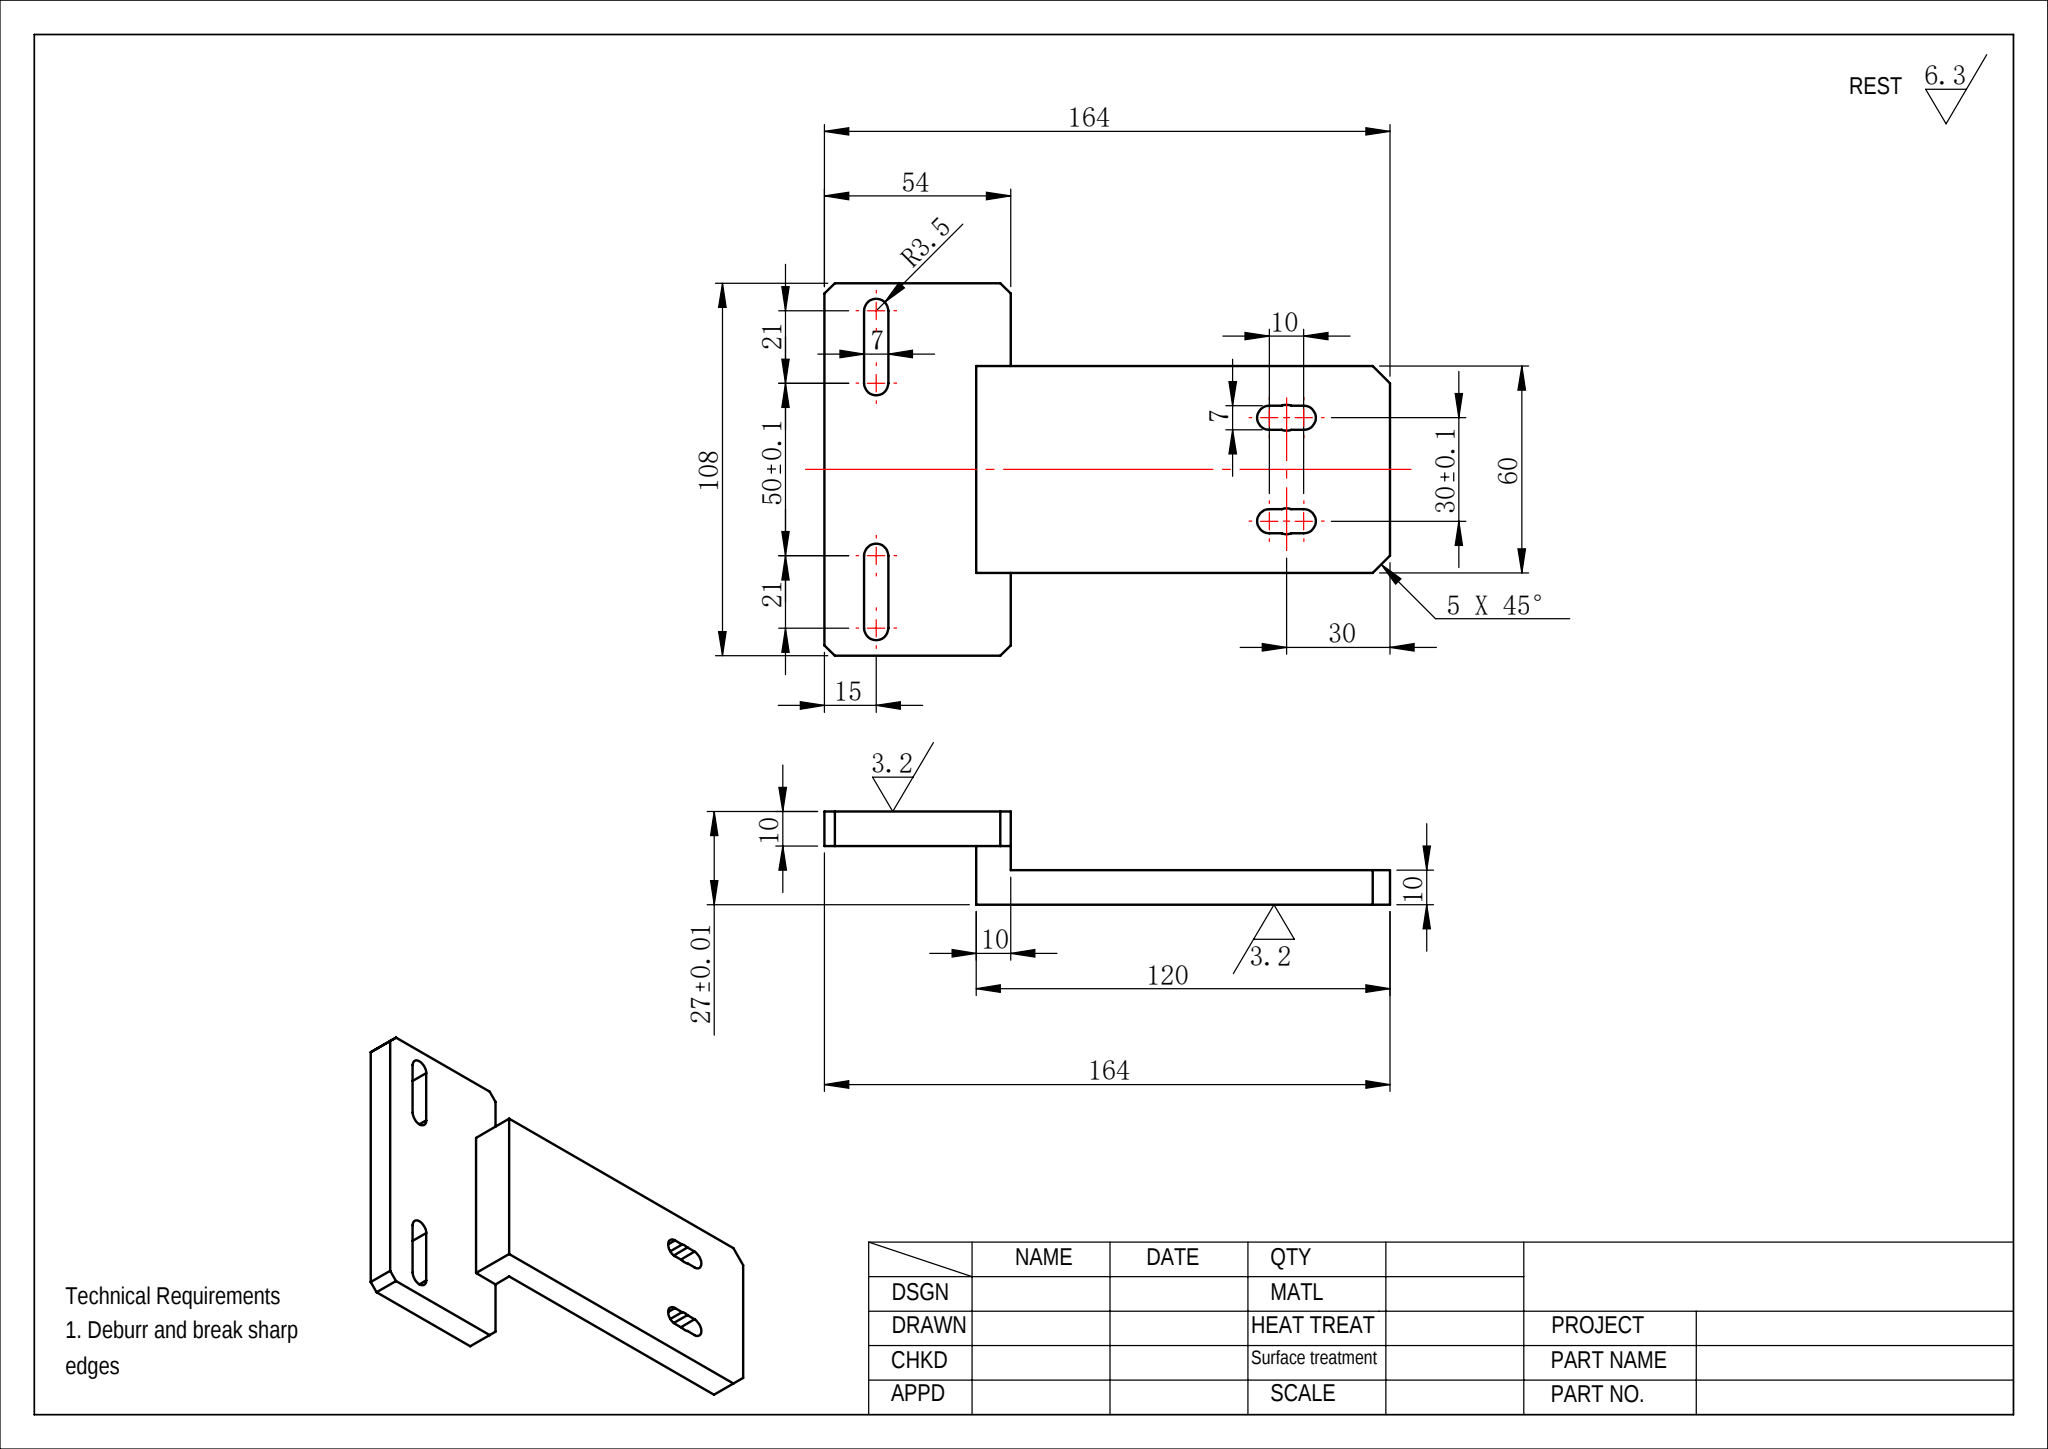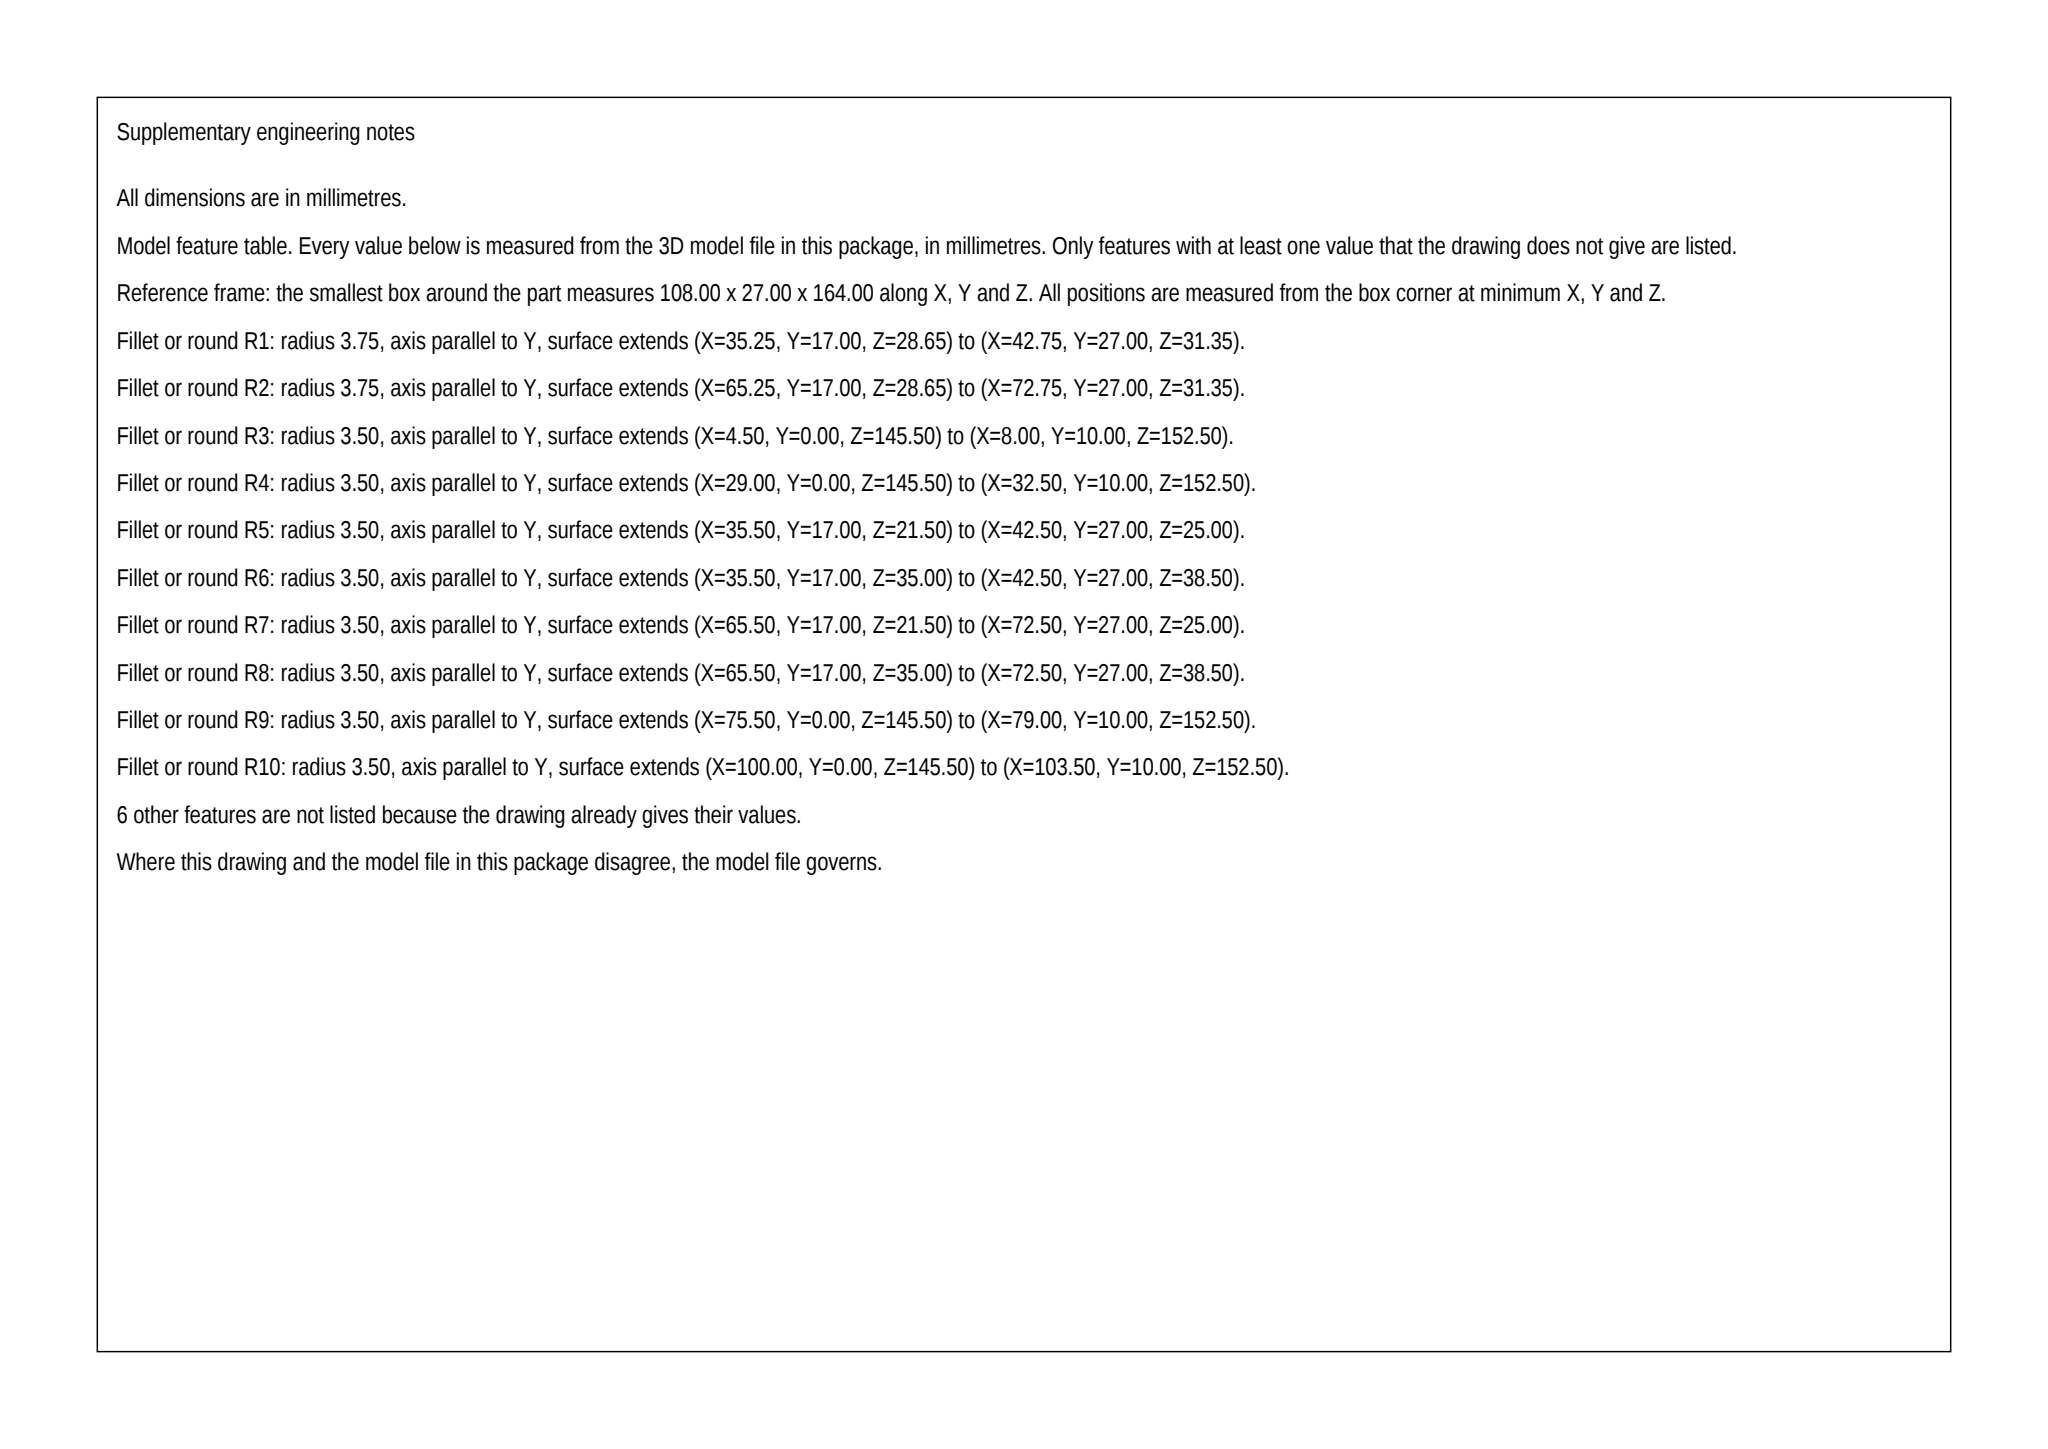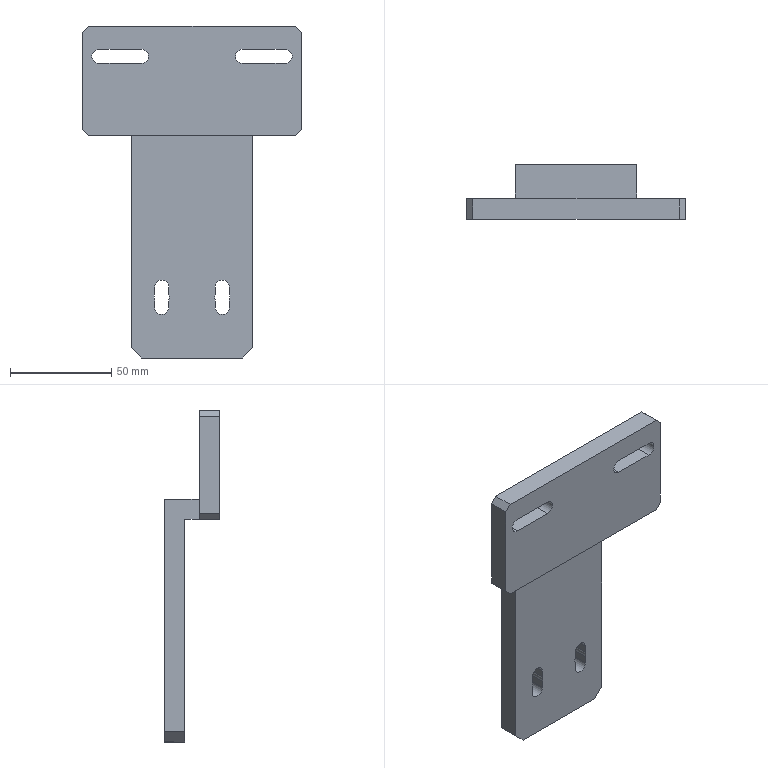Part | SolidWorks | mm | 1 solid | 44 faces | box 108 x 27 x 164 mm | volume 128193 mm3 | plane 30 | cylinder 14 | commonest cylinder face diameters 7 x10 7.5 x4
build123d program:
from build123d import *

# Parameters (mm, degrees)
SKETCH1_W          = 110
SKETCH1_H          = 10
EXTRUDE1_DEPTH     = 54
CUT_EXTRUDE1_DEPTH = 123.947
SKETCH3_W          = 10.185
SKETCH3_H          = 60.979
SKETCH3_W_2        = 12.302
SKETCH3_H_2        = 66.27
CUT_EXTRUDE2_DEPTH = 123.947
SKETCH4_W          = 60
SKETCH4_H          = 10
EXTRUDE2_DEPTH     = 17
SKETCH5_W          = 60
SKETCH5_H          = 10
EXTRUDE3_DEPTH     = 110
CUT_EXTRUDE3_DEPTH = 158.194
CHAMFER1_SIZE      = 5
CHAMFER2_SIZE      = 3


with BuildPart() as part:
    # Sketch1 → Extrude1 (new body)
    with BuildSketch(Plane.XY):
        with Locations((55, 5)):
            Rectangle(SKETCH1_W, SKETCH1_H)
    extrude(amount=EXTRUDE1_DEPTH)

    # Sketch2 → Cut-Extrude1 (cut, through all)
    with BuildSketch(Plane.XZ):
        with BuildLine():
            Line((9, 42.5), (30, 42.5))
            ThreePointArc((30, 42.5), (33.5, 39), (30, 35.5))
            Line((30, 35.5), (9, 35.5))
            ThreePointArc((9, 35.5), (5.5, 39), (9, 42.5))
        make_face()
        with BuildLine():
            Line((80, 42.5), (101, 42.5))
            ThreePointArc((101, 42.5), (104.5, 39), (101, 35.5))
            Line((101, 35.5), (80, 35.5))
            ThreePointArc((80, 35.5), (76.5, 39), (80, 42.5))
        make_face()
    extrude(amount=-CUT_EXTRUDE1_DEPTH, mode=Mode.SUBTRACT)

    # Sketch3 → Cut-Extrude2 (cut, through all)
    with BuildSketch(Plane(origin=(0, 10, 0), x_dir=(1, 0, 0), z_dir=(0, 1, 0))):
        with Locations((114.093, -27.066)):
            Rectangle(SKETCH3_W, SKETCH3_H)
        with Locations((-5.151, -24.421)):
            Rectangle(SKETCH3_W_2, SKETCH3_H_2)
    extrude(amount=-CUT_EXTRUDE2_DEPTH, mode=Mode.SUBTRACT)

    # Sketch4 → Extrude2 (add)
    with BuildSketch(Plane(origin=(0, 10, 0), x_dir=(1, 0, 0), z_dir=(0, 1, 0))):
        with Locations((55, -5)):
            Rectangle(SKETCH4_W, SKETCH4_H)
    extrude(amount=EXTRUDE2_DEPTH)

    # Sketch5 → Extrude3 (add)
    with BuildSketch(Plane(origin=(0, 0, 0), x_dir=(-1, 0, 0), z_dir=(0, 0, -1))):
        with Locations((-55, 22)):
            Rectangle(SKETCH5_W, SKETCH5_H)
    extrude(amount=EXTRUDE3_DEPTH)

    # Sketch6 → Cut-Extrude3 (cut, through all)
    with BuildSketch(Plane(origin=(0, 27, 0), x_dir=(1, 0, 0), z_dir=(0, 1, 0))):
        with BuildLine():
            Line((66.5, 81.346), (66.5, 85))
            ThreePointArc((66.5, 85), (70, 88.5), (73.5, 85))
            Line((73.5, 85), (73.5, 81.346))
            ThreePointArc((73.5, 81.346), (73.75, 80), (73.5, 78.654))
            Line((73.5, 78.654), (73.5, 75))
            ThreePointArc((73.5, 75), (70, 71.5), (66.5, 75))
            Line((66.5, 75), (66.5, 78.654))
            ThreePointArc((66.5, 78.654), (66.25, 80), (66.5, 81.346))
        make_face()
        with BuildLine():
            Line((36.5, 75), (36.5, 78.654))
            ThreePointArc((36.5, 78.654), (36.25, 80), (36.5, 81.346))
            Line((36.5, 81.346), (36.5, 85))
            ThreePointArc((36.5, 85), (40, 88.5), (43.5, 85))
            Line((43.5, 85), (43.5, 81.346))
            ThreePointArc((43.5, 81.346), (43.75, 80), (43.5, 78.654))
            Line((43.5, 78.654), (43.5, 75))
            ThreePointArc((43.5, 75), (40, 71.5), (36.5, 75))
        make_face()
    extrude(amount=-CUT_EXTRUDE3_DEPTH, mode=Mode.SUBTRACT)

    # Chamfer1
    chamfer1_edges = [part.edges().sort_by_distance(p)[0] for p in [
        (25, 22, -110),
        (85, 22, -110),
    ]]
    chamfer(chamfer1_edges, length=CHAMFER1_SIZE)

    # Chamfer2
    chamfer2_edges = [part.edges().sort_by_distance(p)[0] for p in [
        (1, 5, 54),
        (1, 5, 0),
        (109, 5, 54),
        (109, 5, 0),
    ]]
    chamfer(chamfer2_edges, length=CHAMFER2_SIZE)


solid = part.part